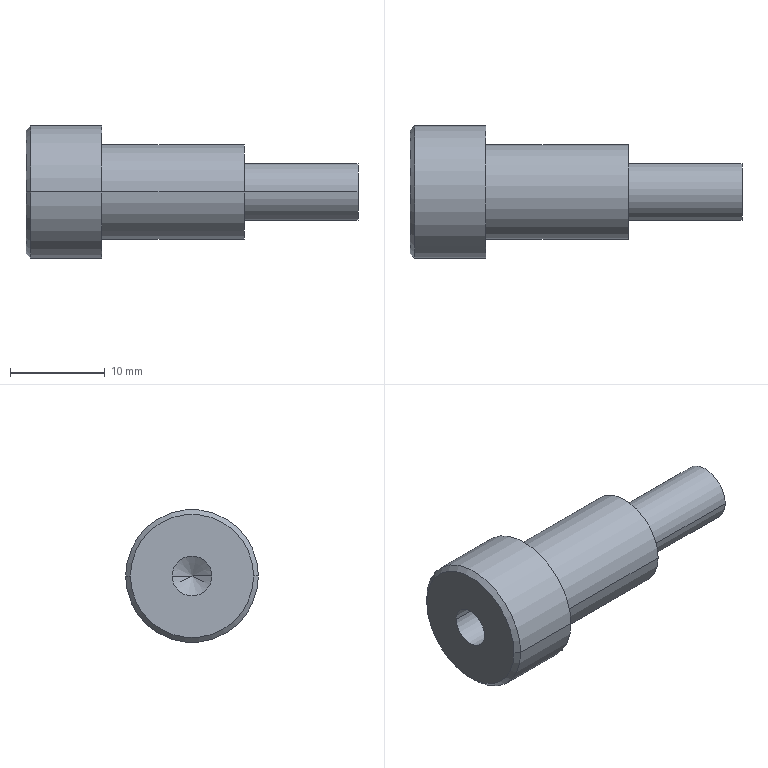Component | SolidWorks | ClampingArm2-1_A74-1 | 1 solid | 20 faces | box 35 x 14 x 14 mm | volume 2528 mm3 | cylinder 10 | cone 6 | plane 4 | commonest cylinder face diameters 2.5 x2 6 x2 4.2 x2 10 x2 14 x2 | material S45C
build123d program:
from build123d import *

# Parameters (mm, degrees)
SKETCH1_R             = 7
BOSS_EXTRUDE1_DEPTH   = 4
CHAMFER1_SIZE         = 0.5
SKETCH4_R             = 5
BOSS_EXTRUDE2_DEPTH   = 15
M5_TAPPED_HOLE1_D     = 4.2
M5_TAPPED_HOLE1_DEPTH = 12.4
M5_TAPPED_HOLE1_TIP   = 1.262
SKETCH7_R             = 3
BOSS_EXTRUDE3_DEPTH   = 12
M3_TAPPED_HOLE1_D     = 2.5
M3_TAPPED_HOLE1_DEPTH = 7.5
M3_TAPPED_HOLE1_TIP   = 0.7511


with BuildPart() as part:
    # Sketch1 → Boss-Extrude1 (new, symmetric)
    with BuildSketch(Plane(origin=(0, 0, 0), x_dir=(0, 0, -1), z_dir=(1, 0, 0))):
        Circle(SKETCH1_R)
    extrude(amount=BOSS_EXTRUDE1_DEPTH, both=True)

    # Chamfer1
    chamfer1_edges = [part.edges().sort_by_distance(p)[0] for p in [
        (-4, 0, 7),
    ]]
    chamfer(chamfer1_edges, length=CHAMFER1_SIZE)

    # Sketch4 → Boss-Extrude2 (add)
    with BuildSketch(Plane(origin=(4, 0, 0), x_dir=(0, 0, -1), z_dir=(1, 0, 0))):
        Circle(SKETCH4_R)
    extrude(amount=BOSS_EXTRUDE2_DEPTH)

    # M5 Tapped Hole1
    with Locations(Plane.ZY.offset(4)):
        with Locations((0, 0)):
            Hole(M5_TAPPED_HOLE1_D / 2, depth=M5_TAPPED_HOLE1_DEPTH)
            with Locations((0, 0, -(M5_TAPPED_HOLE1_DEPTH + M5_TAPPED_HOLE1_TIP / 2))):  # 118° drill point
                Cone(0, M5_TAPPED_HOLE1_D / 2, M5_TAPPED_HOLE1_TIP, mode=Mode.SUBTRACT)

    # Sketch7 → Boss-Extrude3 (add)
    with BuildSketch(Plane(origin=(19, 0, 0), x_dir=(0, 0, -1), z_dir=(1, 0, 0))):
        Circle(SKETCH7_R)
    extrude(amount=BOSS_EXTRUDE3_DEPTH)

    # M3 Tapped Hole1
    with Locations(Plane(origin=(31, 0, 0), x_dir=(0, 0, -1), z_dir=(1, 0, 0))):
        with Locations((0, 0)):
            Hole(M3_TAPPED_HOLE1_D / 2, depth=M3_TAPPED_HOLE1_DEPTH)
            with Locations((0, 0, -(M3_TAPPED_HOLE1_DEPTH + M3_TAPPED_HOLE1_TIP / 2))):  # 118° drill point
                Cone(0, M3_TAPPED_HOLE1_D / 2, M3_TAPPED_HOLE1_TIP, mode=Mode.SUBTRACT)


solid = part.part

# Placed as in the assembly
solid = solid.moved(Location((-33.551, 66.046, -22.5), (0, 0, 0)))
STEP:
#1=CARTESIAN_POINT('',(-0.3957,2.551,-0.8858));
#2=VERTEX_POINT('',#1);
#3=CARTESIAN_POINT('',(-0.3957,2.649,-0.8858));
#4=VERTEX_POINT('',#3);
#5=CARTESIAN_POINT('',(-0.3957,2.6,-0.8858));
#6=DIRECTION('',(1.,0.,-0.));
#7=DIRECTION('',(0.,1.,-0.0003333));
#8=AXIS2_PLACEMENT_3D('',#5,#6,#7);
#9=CIRCLE('',#8,0.04921);
#10=EDGE_CURVE('',#2,#4,#9,.T.);
#11=ORIENTED_EDGE('',*,*,#10,.F.);
#12=CARTESIAN_POINT('',(-0.1004,2.551,-0.8858));
#13=VERTEX_POINT('',#12);
#14=CARTESIAN_POINT('',(-0.1004,2.551,-0.8858));
#15=DIRECTION('',(1.,0.,-0.));
#16=VECTOR('',#15,39.37);
#17=LINE('',#14,#16);
#18=EDGE_CURVE('',#2,#13,#17,.T.);
#19=ORIENTED_EDGE('',*,*,#18,.T.);
#20=CARTESIAN_POINT('',(-0.1004,2.649,-0.8858));
#21=VERTEX_POINT('',#20);
#22=CARTESIAN_POINT('',(-0.1004,2.6,-0.8858));
#23=DIRECTION('',(1.,0.,-0.));
#24=DIRECTION('',(0.,1.,-0.0003333));
#25=AXIS2_PLACEMENT_3D('',#22,#23,#24);
#26=CIRCLE('',#25,0.04921);
#27=EDGE_CURVE('',#13,#21,#26,.T.);
#28=ORIENTED_EDGE('',*,*,#27,.T.);
#29=CARTESIAN_POINT('',(-0.1004,2.649,-0.8858));
#30=DIRECTION('',(1.,0.,-0.));
#31=VECTOR('',#30,39.37);
#32=LINE('',#29,#31);
#33=EDGE_CURVE('',#4,#21,#32,.T.);
#34=ORIENTED_EDGE('',*,*,#33,.F.);
#35=EDGE_LOOP('',(#11,#19,#28,#34));
#36=FACE_OUTER_BOUND('',#35,.T.);
#37=CARTESIAN_POINT('',(-0.1004,2.6,-0.8858));
#38=DIRECTION('',(1.,0.,-0.));
#39=DIRECTION('',(0.,1.,-0.0003333));
#40=AXIS2_PLACEMENT_3D('',#37,#38,#39);
#41=CYLINDRICAL_SURFACE('',#40,0.04921);
#42=ADVANCED_FACE('',(#36),#41,.F.);
#43=CARTESIAN_POINT('',(-0.4253,2.6,-0.8858));
#44=VERTEX_POINT('',#43);
#45=CARTESIAN_POINT('',(-0.3957,2.649,-0.8858));
#46=DIRECTION('',(0.515,0.8572,-0.0002857));
#47=VECTOR('',#46,39.37);
#48=LINE('',#45,#47);
#49=EDGE_CURVE('',#44,#4,#48,.T.);
#50=ORIENTED_EDGE('',*,*,#49,.F.);
#51=CARTESIAN_POINT('',(-0.3957,2.551,-0.8858));
#52=DIRECTION('',(0.515,-0.8572,0.0002857));
#53=VECTOR('',#52,39.37);
#54=LINE('',#51,#53);
#55=EDGE_CURVE('',#44,#2,#54,.T.);
#56=ORIENTED_EDGE('',*,*,#55,.T.);
#57=ORIENTED_EDGE('',*,*,#10,.T.);
#58=EDGE_LOOP('',(#50,#56,#57));
#59=FACE_OUTER_BOUND('',#58,.T.);
#60=CARTESIAN_POINT('',(-0.3957,2.6,-0.8858));
#61=DIRECTION('',(1.,0.,-0.));
#62=DIRECTION('',(0.,1.,-0.0003333));
#63=AXIS2_PLACEMENT_3D('',#60,#61,#62);
#64=CONICAL_SURFACE('',#63,0.04921,1.03);
#65=ADVANCED_FACE('',(#59),#64,.F.);
#66=CARTESIAN_POINT('',(-0.1004,2.718,-0.8859));
#67=VERTEX_POINT('',#66);
#68=CARTESIAN_POINT('',(-0.1004,2.482,-0.8858));
#69=VERTEX_POINT('',#68);
#70=CARTESIAN_POINT('',(-0.1004,2.6,-0.8858));
#71=DIRECTION('',(1.,0.,-0.));
#72=DIRECTION('',(0.,1.,-0.0003333));
#73=AXIS2_PLACEMENT_3D('',#70,#71,#72);
#74=CIRCLE('',#73,0.1181);
#75=EDGE_CURVE('',#67,#69,#74,.T.);
#76=ORIENTED_EDGE('',*,*,#75,.F.);
#77=CARTESIAN_POINT('',(-0.5729,2.718,-0.8859));
#78=VERTEX_POINT('',#77);
#79=CARTESIAN_POINT('',(-0.1004,2.718,-0.8859));
#80=DIRECTION('',(-1.,-0.,0.));
#81=VECTOR('',#80,39.37);
#82=LINE('',#79,#81);
#83=EDGE_CURVE('',#67,#78,#82,.T.);
#84=ORIENTED_EDGE('',*,*,#83,.T.);
#85=CARTESIAN_POINT('',(-0.5729,2.482,-0.8858));
#86=VERTEX_POINT('',#85);
#87=CARTESIAN_POINT('',(-0.5729,2.6,-0.8858));
#88=DIRECTION('',(1.,0.,-0.));
#89=DIRECTION('',(0.,1.,-0.0003333));
#90=AXIS2_PLACEMENT_3D('',#87,#88,#89);
#91=CIRCLE('',#90,0.1181);
#92=EDGE_CURVE('',#78,#86,#91,.T.);
#93=ORIENTED_EDGE('',*,*,#92,.T.);
#94=CARTESIAN_POINT('',(-0.1004,2.482,-0.8858));
#95=DIRECTION('',(-1.,-0.,0.));
#96=VECTOR('',#95,39.37);
#97=LINE('',#94,#96);
#98=EDGE_CURVE('',#69,#86,#97,.T.);
#99=ORIENTED_EDGE('',*,*,#98,.F.);
#100=EDGE_LOOP('',(#76,#84,#93,#99));
#101=FACE_OUTER_BOUND('',#100,.T.);
#102=CARTESIAN_POINT('',(-0.1004,2.6,-0.8858));
#103=DIRECTION('',(-1.,-0.,0.));
#104=DIRECTION('',(0.,-1.,0.0003333));
#105=AXIS2_PLACEMENT_3D('',#102,#103,#104);
#106=CYLINDRICAL_SURFACE('',#105,0.1181);
#107=ADVANCED_FACE('',(#101),#106,.T.);
#108=CARTESIAN_POINT('',(-0.9902,2.683,-0.8859));
#109=VERTEX_POINT('',#108);
#110=CARTESIAN_POINT('',(-0.9902,2.518,-0.8858));
#111=VERTEX_POINT('',#110);
#112=CARTESIAN_POINT('',(-0.9902,2.6,-0.8858));
#113=DIRECTION('',(-1.,-0.,0.));
#114=DIRECTION('',(0.,-1.,0.0003333));
#115=AXIS2_PLACEMENT_3D('',#112,#113,#114);
#116=CIRCLE('',#115,0.08268);
#117=EDGE_CURVE('',#109,#111,#116,.T.);
#118=ORIENTED_EDGE('',*,*,#117,.F.);
#119=CARTESIAN_POINT('',(-1.478,2.683,-0.8859));
#120=VERTEX_POINT('',#119);
#121=CARTESIAN_POINT('',(-1.478,2.683,-0.8859));
#122=DIRECTION('',(-1.,-0.,0.));
#123=VECTOR('',#122,39.37);
#124=LINE('',#121,#123);
#125=EDGE_CURVE('',#109,#120,#124,.T.);
#126=ORIENTED_EDGE('',*,*,#125,.T.);
#127=CARTESIAN_POINT('',(-1.478,2.518,-0.8858));
#128=VERTEX_POINT('',#127);
#129=CARTESIAN_POINT('',(-1.478,2.6,-0.8858));
#130=DIRECTION('',(-1.,-0.,0.));
#131=DIRECTION('',(0.,-1.,0.0003333));
#132=AXIS2_PLACEMENT_3D('',#129,#130,#131);
#133=CIRCLE('',#132,0.08268);
#134=EDGE_CURVE('',#120,#128,#133,.T.);
#135=ORIENTED_EDGE('',*,*,#134,.T.);
#136=CARTESIAN_POINT('',(-1.478,2.518,-0.8858));
#137=DIRECTION('',(-1.,-0.,0.));
#138=VECTOR('',#137,39.37);
#139=LINE('',#136,#138);
#140=EDGE_CURVE('',#111,#128,#139,.T.);
#141=ORIENTED_EDGE('',*,*,#140,.F.);
#142=EDGE_LOOP('',(#118,#126,#135,#141));
#143=FACE_OUTER_BOUND('',#142,.T.);
#144=CARTESIAN_POINT('',(-1.478,2.6,-0.8858));
#145=DIRECTION('',(-1.,-0.,0.));
#146=DIRECTION('',(0.,-1.,0.0003333));
#147=AXIS2_PLACEMENT_3D('',#144,#145,#146);
#148=CYLINDRICAL_SURFACE('',#147,0.08268);
#149=ADVANCED_FACE('',(#143),#148,.F.);
#150=CARTESIAN_POINT('',(-0.9405,2.6,-0.8858));
#151=VERTEX_POINT('',#150);
#152=CARTESIAN_POINT('',(-0.9902,2.518,-0.8858));
#153=DIRECTION('',(-0.515,-0.8572,0.0002857));
#154=VECTOR('',#153,39.37);
#155=LINE('',#152,#154);
#156=EDGE_CURVE('',#151,#111,#155,.T.);
#157=ORIENTED_EDGE('',*,*,#156,.F.);
#158=CARTESIAN_POINT('',(-0.9902,2.683,-0.8859));
#159=DIRECTION('',(-0.515,0.8572,-0.0002857));
#160=VECTOR('',#159,39.37);
#161=LINE('',#158,#160);
#162=EDGE_CURVE('',#151,#109,#161,.T.);
#163=ORIENTED_EDGE('',*,*,#162,.T.);
#164=ORIENTED_EDGE('',*,*,#117,.T.);
#165=EDGE_LOOP('',(#157,#163,#164));
#166=FACE_OUTER_BOUND('',#165,.T.);
#167=CARTESIAN_POINT('',(-0.9902,2.6,-0.8858));
#168=DIRECTION('',(-1.,-0.,0.));
#169=DIRECTION('',(0.,-1.,0.0003333));
#170=AXIS2_PLACEMENT_3D('',#167,#168,#169);
#171=CONICAL_SURFACE('',#170,0.08268,1.03);
#172=ADVANCED_FACE('',(#166),#171,.F.);
#173=CARTESIAN_POINT('',(-0.5729,2.797,-0.8859));
#174=VERTEX_POINT('',#173);
#175=CARTESIAN_POINT('',(-0.5729,2.403,-0.8858));
#176=VERTEX_POINT('',#175);
#177=CARTESIAN_POINT('',(-0.5729,2.6,-0.8858));
#178=DIRECTION('',(1.,0.,-0.));
#179=DIRECTION('',(0.,1.,-0.0003333));
#180=AXIS2_PLACEMENT_3D('',#177,#178,#179);
#181=CIRCLE('',#180,0.1969);
#182=EDGE_CURVE('',#174,#176,#181,.T.);
#183=ORIENTED_EDGE('',*,*,#182,.F.);
#184=CARTESIAN_POINT('',(-1.163,2.797,-0.8859));
#185=VERTEX_POINT('',#184);
#186=CARTESIAN_POINT('',(-0.5729,2.797,-0.8859));
#187=DIRECTION('',(-1.,-0.,0.));
#188=VECTOR('',#187,39.37);
#189=LINE('',#186,#188);
#190=EDGE_CURVE('',#174,#185,#189,.T.);
#191=ORIENTED_EDGE('',*,*,#190,.T.);
#192=CARTESIAN_POINT('',(-1.163,2.403,-0.8858));
#193=VERTEX_POINT('',#192);
#194=CARTESIAN_POINT('',(-1.163,2.6,-0.8858));
#195=DIRECTION('',(1.,0.,-0.));
#196=DIRECTION('',(0.,1.,-0.0003333));
#197=AXIS2_PLACEMENT_3D('',#194,#195,#196);
#198=CIRCLE('',#197,0.1969);
#199=EDGE_CURVE('',#185,#193,#198,.T.);
#200=ORIENTED_EDGE('',*,*,#199,.T.);
#201=CARTESIAN_POINT('',(-0.5729,2.403,-0.8858));
#202=DIRECTION('',(-1.,-0.,0.));
#203=VECTOR('',#202,39.37);
#204=LINE('',#201,#203);
#205=EDGE_CURVE('',#176,#193,#204,.T.);
#206=ORIENTED_EDGE('',*,*,#205,.F.);
#207=EDGE_LOOP('',(#183,#191,#200,#206));
#208=FACE_OUTER_BOUND('',#207,.T.);
#209=CARTESIAN_POINT('',(-0.5729,2.6,-0.8858));
#210=DIRECTION('',(-1.,-0.,0.));
#211=DIRECTION('',(0.,-1.,0.0003333));
#212=AXIS2_PLACEMENT_3D('',#209,#210,#211);
#213=CYLINDRICAL_SURFACE('',#212,0.1969);
#214=ADVANCED_FACE('',(#208),#213,.T.);
#215=CARTESIAN_POINT('',(-1.478,2.344,-0.8857));
#216=VERTEX_POINT('',#215);
#217=CARTESIAN_POINT('',(-1.478,2.856,-0.8859));
#218=VERTEX_POINT('',#217);
#219=CARTESIAN_POINT('',(-1.478,2.6,-0.8858));
#220=DIRECTION('',(-1.,-0.,0.));
#221=DIRECTION('',(0.,1.,-0.0003333));
#222=AXIS2_PLACEMENT_3D('',#219,#220,#221);
#223=CIRCLE('',#222,0.2559);
#224=EDGE_CURVE('',#216,#218,#223,.T.);
#225=ORIENTED_EDGE('',*,*,#224,.F.);
#226=CARTESIAN_POINT('',(-1.459,2.325,-0.8857));
#227=VERTEX_POINT('',#226);
#228=CARTESIAN_POINT('',(-1.459,2.325,-0.8857));
#229=DIRECTION('',(0.7071,-0.7071,0.0002357));
#230=VECTOR('',#229,39.37);
#231=LINE('',#228,#230);
#232=EDGE_CURVE('',#216,#227,#231,.T.);
#233=ORIENTED_EDGE('',*,*,#232,.T.);
#234=CARTESIAN_POINT('',(-1.459,2.876,-0.8859));
#235=VERTEX_POINT('',#234);
#236=CARTESIAN_POINT('',(-1.459,2.6,-0.8858));
#237=DIRECTION('',(1.,0.,-0.));
#238=DIRECTION('',(0.,1.,-0.0003333));
#239=AXIS2_PLACEMENT_3D('',#236,#237,#238);
#240=CIRCLE('',#239,0.2756);
#241=EDGE_CURVE('',#235,#227,#240,.T.);
#242=ORIENTED_EDGE('',*,*,#241,.F.);
#243=CARTESIAN_POINT('',(-1.459,2.876,-0.8859));
#244=DIRECTION('',(0.7071,0.7071,-0.0002357));
#245=VECTOR('',#244,39.37);
#246=LINE('',#243,#245);
#247=EDGE_CURVE('',#218,#235,#246,.T.);
#248=ORIENTED_EDGE('',*,*,#247,.F.);
#249=EDGE_LOOP('',(#225,#233,#242,#248));
#250=FACE_OUTER_BOUND('',#249,.T.);
#251=CARTESIAN_POINT('',(-1.459,2.6,-0.8858));
#252=DIRECTION('',(1.,0.,-0.));
#253=DIRECTION('',(0.,1.,-0.0003333));
#254=AXIS2_PLACEMENT_3D('',#251,#252,#253);
#255=CONICAL_SURFACE('',#254,0.2756,0.7854);
#256=ADVANCED_FACE('',(#250),#255,.T.);
#257=CARTESIAN_POINT('',(-1.163,2.876,-0.8859));
#258=VERTEX_POINT('',#257);
#259=CARTESIAN_POINT('',(-1.163,2.325,-0.8857));
#260=VERTEX_POINT('',#259);
#261=CARTESIAN_POINT('',(-1.163,2.6,-0.8858));
#262=DIRECTION('',(1.,0.,-0.));
#263=DIRECTION('',(0.,1.,-0.0003333));
#264=AXIS2_PLACEMENT_3D('',#261,#262,#263);
#265=CIRCLE('',#264,0.2756);
#266=EDGE_CURVE('',#258,#260,#265,.T.);
#267=ORIENTED_EDGE('',*,*,#266,.F.);
#268=CARTESIAN_POINT('',(-1.163,2.876,-0.8859));
#269=DIRECTION('',(-1.,-0.,0.));
#270=VECTOR('',#269,39.37);
#271=LINE('',#268,#270);
#272=EDGE_CURVE('',#258,#235,#271,.T.);
#273=ORIENTED_EDGE('',*,*,#272,.T.);
#274=ORIENTED_EDGE('',*,*,#241,.T.);
#275=CARTESIAN_POINT('',(-1.163,2.325,-0.8857));
#276=DIRECTION('',(-1.,-0.,0.));
#277=VECTOR('',#276,39.37);
#278=LINE('',#275,#277);
#279=EDGE_CURVE('',#260,#227,#278,.T.);
#280=ORIENTED_EDGE('',*,*,#279,.F.);
#281=EDGE_LOOP('',(#267,#273,#274,#280));
#282=FACE_OUTER_BOUND('',#281,.T.);
#283=CARTESIAN_POINT('',(-1.163,2.6,-0.8858));
#284=DIRECTION('',(-1.,-0.,0.));
#285=DIRECTION('',(0.,-1.,0.0003333));
#286=AXIS2_PLACEMENT_3D('',#283,#284,#285);
#287=CYLINDRICAL_SURFACE('',#286,0.2756);
#288=ADVANCED_FACE('',(#282),#287,.T.);
#289=ORIENTED_EDGE('',*,*,#272,.F.);
#290=CARTESIAN_POINT('',(-1.163,2.6,-0.8858));
#291=DIRECTION('',(1.,0.,-0.));
#292=DIRECTION('',(0.,1.,-0.0003333));
#293=AXIS2_PLACEMENT_3D('',#290,#291,#292);
#294=CIRCLE('',#293,0.2756);
#295=EDGE_CURVE('',#260,#258,#294,.T.);
#296=ORIENTED_EDGE('',*,*,#295,.F.);
#297=ORIENTED_EDGE('',*,*,#279,.T.);
#298=CARTESIAN_POINT('',(-1.459,2.6,-0.8858));
#299=DIRECTION('',(1.,0.,-0.));
#300=DIRECTION('',(0.,1.,-0.0003333));
#301=AXIS2_PLACEMENT_3D('',#298,#299,#300);
#302=CIRCLE('',#301,0.2756);
#303=EDGE_CURVE('',#227,#235,#302,.T.);
#304=ORIENTED_EDGE('',*,*,#303,.T.);
#305=EDGE_LOOP('',(#289,#296,#297,#304));
#306=FACE_OUTER_BOUND('',#305,.T.);
#307=CARTESIAN_POINT('',(-1.163,2.6,-0.8858));
#308=DIRECTION('',(-1.,-0.,0.));
#309=DIRECTION('',(0.,-1.,0.0003333));
#310=AXIS2_PLACEMENT_3D('',#307,#308,#309);
#311=CYLINDRICAL_SURFACE('',#310,0.2756);
#312=ADVANCED_FACE('',(#306),#311,.T.);
#313=CARTESIAN_POINT('',(-1.163,2.6,-0.8858));
#314=DIRECTION('',(1.,0.,-0.));
#315=DIRECTION('',(0.,1.,-0.0003333));
#316=AXIS2_PLACEMENT_3D('',#313,#314,#315);
#317=CIRCLE('',#316,0.1969);
#318=EDGE_CURVE('',#193,#185,#317,.T.);
#319=ORIENTED_EDGE('',*,*,#318,.F.);
#320=ORIENTED_EDGE('',*,*,#199,.F.);
#321=EDGE_LOOP('',(#319,#320));
#322=FACE_BOUND('',#321,.T.);
#323=ORIENTED_EDGE('',*,*,#295,.T.);
#324=ORIENTED_EDGE('',*,*,#266,.T.);
#325=EDGE_LOOP('',(#323,#324));
#326=FACE_OUTER_BOUND('',#325,.T.);
#327=CARTESIAN_POINT('',(-1.163,2.6,-0.8858));
#328=DIRECTION('',(1.,0.,-0.));
#329=DIRECTION('',(-0.,1.,-0.0003333));
#330=AXIS2_PLACEMENT_3D('',#327,#328,#329);
#331=PLANE('',#330);
#332=ADVANCED_FACE('',(#322,#326),#331,.T.);
#333=CARTESIAN_POINT('',(-1.478,2.6,-0.8858));
#334=DIRECTION('',(-1.,-0.,0.));
#335=DIRECTION('',(0.,-1.,0.0003333));
#336=AXIS2_PLACEMENT_3D('',#333,#334,#335);
#337=CIRCLE('',#336,0.08268);
#338=EDGE_CURVE('',#128,#120,#337,.T.);
#339=ORIENTED_EDGE('',*,*,#338,.F.);
#340=ORIENTED_EDGE('',*,*,#134,.F.);
#341=EDGE_LOOP('',(#339,#340));
#342=FACE_BOUND('',#341,.T.);
#343=CARTESIAN_POINT('',(-1.478,2.6,-0.8858));
#344=DIRECTION('',(-1.,-0.,0.));
#345=DIRECTION('',(0.,1.,-0.0003333));
#346=AXIS2_PLACEMENT_3D('',#343,#344,#345);
#347=CIRCLE('',#346,0.2559);
#348=EDGE_CURVE('',#218,#216,#347,.T.);
#349=ORIENTED_EDGE('',*,*,#348,.T.);
#350=ORIENTED_EDGE('',*,*,#224,.T.);
#351=EDGE_LOOP('',(#349,#350));
#352=FACE_OUTER_BOUND('',#351,.T.);
#353=CARTESIAN_POINT('',(-1.478,2.6,-0.8858));
#354=DIRECTION('',(1.,0.,-0.));
#355=DIRECTION('',(-0.,1.,-0.0003333));
#356=AXIS2_PLACEMENT_3D('',#353,#354,#355);
#357=PLANE('',#356);
#358=ADVANCED_FACE('',(#342,#352),#357,.F.);
#359=ORIENTED_EDGE('',*,*,#232,.F.);
#360=ORIENTED_EDGE('',*,*,#348,.F.);
#361=ORIENTED_EDGE('',*,*,#247,.T.);
#362=ORIENTED_EDGE('',*,*,#303,.F.);
#363=EDGE_LOOP('',(#359,#360,#361,#362));
#364=FACE_OUTER_BOUND('',#363,.T.);
#365=CARTESIAN_POINT('',(-1.459,2.6,-0.8858));
#366=DIRECTION('',(1.,0.,-0.));
#367=DIRECTION('',(0.,1.,-0.0003333));
#368=AXIS2_PLACEMENT_3D('',#365,#366,#367);
#369=CONICAL_SURFACE('',#368,0.2756,0.7854);
#370=ADVANCED_FACE('',(#364),#369,.T.);
#371=ORIENTED_EDGE('',*,*,#190,.F.);
#372=CARTESIAN_POINT('',(-0.5729,2.6,-0.8858));
#373=DIRECTION('',(1.,0.,-0.));
#374=DIRECTION('',(0.,1.,-0.0003333));
#375=AXIS2_PLACEMENT_3D('',#372,#373,#374);
#376=CIRCLE('',#375,0.1969);
#377=EDGE_CURVE('',#176,#174,#376,.T.);
#378=ORIENTED_EDGE('',*,*,#377,.F.);
#379=ORIENTED_EDGE('',*,*,#205,.T.);
#380=ORIENTED_EDGE('',*,*,#318,.T.);
#381=EDGE_LOOP('',(#371,#378,#379,#380));
#382=FACE_OUTER_BOUND('',#381,.T.);
#383=CARTESIAN_POINT('',(-0.5729,2.6,-0.8858));
#384=DIRECTION('',(-1.,-0.,0.));
#385=DIRECTION('',(0.,-1.,0.0003333));
#386=AXIS2_PLACEMENT_3D('',#383,#384,#385);
#387=CYLINDRICAL_SURFACE('',#386,0.1969);
#388=ADVANCED_FACE('',(#382),#387,.T.);
#389=CARTESIAN_POINT('',(-0.5729,2.6,-0.8858));
#390=DIRECTION('',(1.,0.,-0.));
#391=DIRECTION('',(0.,1.,-0.0003333));
#392=AXIS2_PLACEMENT_3D('',#389,#390,#391);
#393=CIRCLE('',#392,0.1181);
#394=EDGE_CURVE('',#86,#78,#393,.T.);
#395=ORIENTED_EDGE('',*,*,#394,.F.);
#396=ORIENTED_EDGE('',*,*,#92,.F.);
#397=EDGE_LOOP('',(#395,#396));
#398=FACE_BOUND('',#397,.T.);
#399=ORIENTED_EDGE('',*,*,#377,.T.);
#400=ORIENTED_EDGE('',*,*,#182,.T.);
#401=EDGE_LOOP('',(#399,#400));
#402=FACE_OUTER_BOUND('',#401,.T.);
#403=CARTESIAN_POINT('',(-0.5729,2.6,-0.8858));
#404=DIRECTION('',(1.,0.,-0.));
#405=DIRECTION('',(-0.,1.,-0.0003333));
#406=AXIS2_PLACEMENT_3D('',#403,#404,#405);
#407=PLANE('',#406);
#408=ADVANCED_FACE('',(#398,#402),#407,.T.);
#409=ORIENTED_EDGE('',*,*,#162,.F.);
#410=ORIENTED_EDGE('',*,*,#156,.T.);
#411=CARTESIAN_POINT('',(-0.9902,2.6,-0.8858));
#412=DIRECTION('',(-1.,-0.,0.));
#413=DIRECTION('',(0.,-1.,0.0003333));
#414=AXIS2_PLACEMENT_3D('',#411,#412,#413);
#415=CIRCLE('',#414,0.08268);
#416=EDGE_CURVE('',#111,#109,#415,.T.);
#417=ORIENTED_EDGE('',*,*,#416,.T.);
#418=EDGE_LOOP('',(#409,#410,#417));
#419=FACE_OUTER_BOUND('',#418,.T.);
#420=CARTESIAN_POINT('',(-0.9902,2.6,-0.8858));
#421=DIRECTION('',(-1.,-0.,0.));
#422=DIRECTION('',(0.,-1.,0.0003333));
#423=AXIS2_PLACEMENT_3D('',#420,#421,#422);
#424=CONICAL_SURFACE('',#423,0.08268,1.03);
#425=ADVANCED_FACE('',(#419),#424,.F.);
#426=ORIENTED_EDGE('',*,*,#125,.F.);
#427=ORIENTED_EDGE('',*,*,#416,.F.);
#428=ORIENTED_EDGE('',*,*,#140,.T.);
#429=ORIENTED_EDGE('',*,*,#338,.T.);
#430=EDGE_LOOP('',(#426,#427,#428,#429));
#431=FACE_OUTER_BOUND('',#430,.T.);
#432=CARTESIAN_POINT('',(-1.478,2.6,-0.8858));
#433=DIRECTION('',(-1.,-0.,0.));
#434=DIRECTION('',(0.,-1.,0.0003333));
#435=AXIS2_PLACEMENT_3D('',#432,#433,#434);
#436=CYLINDRICAL_SURFACE('',#435,0.08268);
#437=ADVANCED_FACE('',(#431),#436,.F.);
#438=ORIENTED_EDGE('',*,*,#83,.F.);
#439=CARTESIAN_POINT('',(-0.1004,2.6,-0.8858));
#440=DIRECTION('',(1.,0.,-0.));
#441=DIRECTION('',(0.,1.,-0.0003333));
#442=AXIS2_PLACEMENT_3D('',#439,#440,#441);
#443=CIRCLE('',#442,0.1181);
#444=EDGE_CURVE('',#69,#67,#443,.T.);
#445=ORIENTED_EDGE('',*,*,#444,.F.);
#446=ORIENTED_EDGE('',*,*,#98,.T.);
#447=ORIENTED_EDGE('',*,*,#394,.T.);
#448=EDGE_LOOP('',(#438,#445,#446,#447));
#449=FACE_OUTER_BOUND('',#448,.T.);
#450=CARTESIAN_POINT('',(-0.1004,2.6,-0.8858));
#451=DIRECTION('',(-1.,-0.,0.));
#452=DIRECTION('',(0.,-1.,0.0003333));
#453=AXIS2_PLACEMENT_3D('',#450,#451,#452);
#454=CYLINDRICAL_SURFACE('',#453,0.1181);
#455=ADVANCED_FACE('',(#449),#454,.T.);
#456=CARTESIAN_POINT('',(-0.1004,2.6,-0.8858));
#457=DIRECTION('',(1.,0.,-0.));
#458=DIRECTION('',(0.,1.,-0.0003333));
#459=AXIS2_PLACEMENT_3D('',#456,#457,#458);
#460=CIRCLE('',#459,0.04921);
#461=EDGE_CURVE('',#21,#13,#460,.T.);
#462=ORIENTED_EDGE('',*,*,#461,.F.);
#463=ORIENTED_EDGE('',*,*,#27,.F.);
#464=EDGE_LOOP('',(#462,#463));
#465=FACE_BOUND('',#464,.T.);
#466=ORIENTED_EDGE('',*,*,#444,.T.);
#467=ORIENTED_EDGE('',*,*,#75,.T.);
#468=EDGE_LOOP('',(#466,#467));
#469=FACE_OUTER_BOUND('',#468,.T.);
#470=CARTESIAN_POINT('',(-0.1004,2.6,-0.8858));
#471=DIRECTION('',(1.,0.,-0.));
#472=DIRECTION('',(-0.,1.,-0.0003333));
#473=AXIS2_PLACEMENT_3D('',#470,#471,#472);
#474=PLANE('',#473);
#475=ADVANCED_FACE('',(#465,#469),#474,.T.);
#476=ORIENTED_EDGE('',*,*,#55,.F.);
#477=ORIENTED_EDGE('',*,*,#49,.T.);
#478=CARTESIAN_POINT('',(-0.3957,2.6,-0.8858));
#479=DIRECTION('',(1.,0.,-0.));
#480=DIRECTION('',(0.,1.,-0.0003333));
#481=AXIS2_PLACEMENT_3D('',#478,#479,#480);
#482=CIRCLE('',#481,0.04921);
#483=EDGE_CURVE('',#4,#2,#482,.T.);
#484=ORIENTED_EDGE('',*,*,#483,.T.);
#485=EDGE_LOOP('',(#476,#477,#484));
#486=FACE_OUTER_BOUND('',#485,.T.);
#487=CARTESIAN_POINT('',(-0.3957,2.6,-0.8858));
#488=DIRECTION('',(1.,0.,-0.));
#489=DIRECTION('',(0.,1.,-0.0003333));
#490=AXIS2_PLACEMENT_3D('',#487,#488,#489);
#491=CONICAL_SURFACE('',#490,0.04921,1.03);
#492=ADVANCED_FACE('',(#486),#491,.F.);
#493=ORIENTED_EDGE('',*,*,#18,.F.);
#494=ORIENTED_EDGE('',*,*,#483,.F.);
#495=ORIENTED_EDGE('',*,*,#33,.T.);
#496=ORIENTED_EDGE('',*,*,#461,.T.);
#497=EDGE_LOOP('',(#493,#494,#495,#496));
#498=FACE_OUTER_BOUND('',#497,.T.);
#499=CARTESIAN_POINT('',(-0.1004,2.6,-0.8858));
#500=DIRECTION('',(1.,0.,-0.));
#501=DIRECTION('',(0.,1.,-0.0003333));
#502=AXIS2_PLACEMENT_3D('',#499,#500,#501);
#503=CYLINDRICAL_SURFACE('',#502,0.04921);
#504=ADVANCED_FACE('',(#498),#503,.F.);
#505=CLOSED_SHELL('',(#42,#65,#107,#149,#172,#214,#256,#288,#312,#332,#358,#370,#388,#408,#425,#437,#455,#475,#492,#504));
#506=MANIFOLD_SOLID_BREP('',#505);
#507=CARTESIAN_POINT('',(0.,0.,0.));
#508=DIRECTION('',(0.,0.,1.));
#509=DIRECTION('',(1.,0.,0.));
#510=AXIS2_PLACEMENT_3D('',#507,#508,#509);
#511=(LENGTH_UNIT()NAMED_UNIT(*)SI_UNIT($,.METRE.));
#512=LENGTH_MEASURE_WITH_UNIT(LENGTH_MEASURE(0.0254),#511);
#513=DIMENSIONAL_EXPONENTS(1.,0.,0.,0.,0.,0.,0.);
#514=(CONVERSION_BASED_UNIT('',#512)LENGTH_UNIT()NAMED_UNIT(#513));
#515=UNCERTAINTY_MEASURE_WITH_UNIT(LENGTH_MEASURE(0.00001),#514,'','');
#516=(NAMED_UNIT(*)PLANE_ANGLE_UNIT()SI_UNIT($,.RADIAN.));
#517=(NAMED_UNIT(*)SI_UNIT($,.STERADIAN.)SOLID_ANGLE_UNIT());
#518=(GEOMETRIC_REPRESENTATION_CONTEXT(3)GLOBAL_UNCERTAINTY_ASSIGNED_CONTEXT((#515))GLOBAL_UNIT_ASSIGNED_CONTEXT((#514,#516,#517))REPRESENTATION_CONTEXT('',''));
#519=ADVANCED_BREP_SHAPE_REPRESENTATION('',(#506,#510),#518);
#520=COLOUR_RGB('',0.7922,0.8196,0.9333);
#521=FILL_AREA_STYLE_COLOUR('',#520);
#522=FILL_AREA_STYLE('',(#521));
#523=SURFACE_STYLE_FILL_AREA(#522);
#524=SURFACE_SIDE_STYLE('',(#523));
#525=SURFACE_STYLE_USAGE(.BOTH.,#524);
#526=PRESENTATION_STYLE_ASSIGNMENT((#525));
#527=STYLED_ITEM('',(#526),#506);
#528=PRESENTATION_LAYER_ASSIGNMENT('','',(#527));
#529=(LENGTH_UNIT()NAMED_UNIT(*)SI_UNIT($,.METRE.));
#530=LENGTH_MEASURE_WITH_UNIT(LENGTH_MEASURE(0.0254),#529);
#531=DIMENSIONAL_EXPONENTS(1.,0.,0.,0.,0.,0.,0.);
#532=(CONVERSION_BASED_UNIT('',#530)LENGTH_UNIT()NAMED_UNIT(#531));
#533=UNCERTAINTY_MEASURE_WITH_UNIT(LENGTH_MEASURE(0.00001),#532,'','');
#534=(NAMED_UNIT(*)PLANE_ANGLE_UNIT()SI_UNIT($,.RADIAN.));
#535=(NAMED_UNIT(*)SI_UNIT($,.STERADIAN.)SOLID_ANGLE_UNIT());
#536=(GEOMETRIC_REPRESENTATION_CONTEXT(3)GLOBAL_UNCERTAINTY_ASSIGNED_CONTEXT((#533))GLOBAL_UNIT_ASSIGNED_CONTEXT((#532,#534,#535))REPRESENTATION_CONTEXT('',''));
#537=MECHANICAL_DESIGN_GEOMETRIC_PRESENTATION_REPRESENTATION('',(#527),#536);